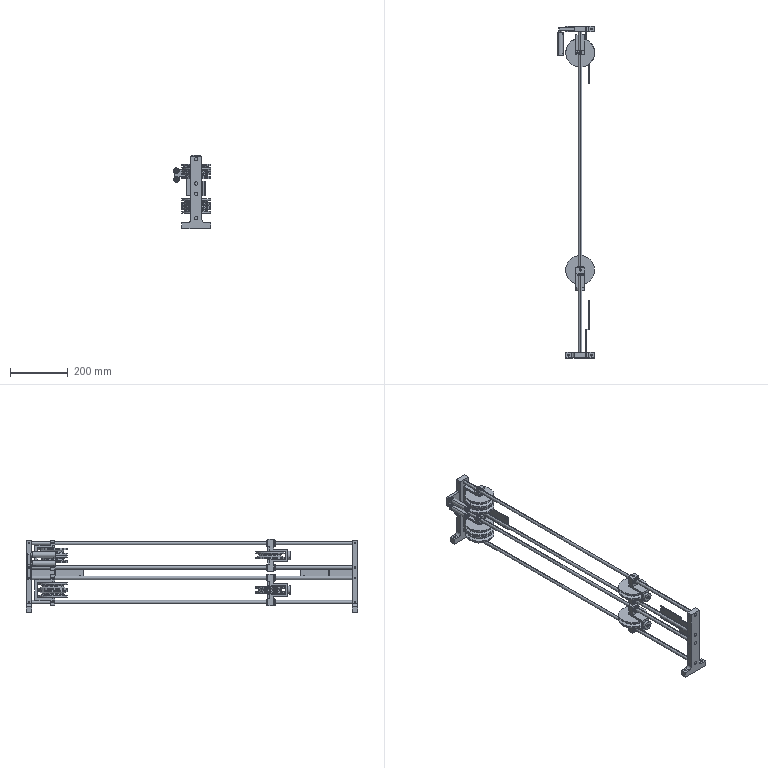Assembly | SolidWorks | mm | 77 component files | 77 solids | 2793 faces | box 129 x 1150 x 253 mm | volume 2246708 mm3 | cylinder 1288 | plane 521 | sphere 448 | torus 400 | cone 72 | spline 64 | commonest cylinder face diameters 1.794 x416 8 x72 12 x52 22 x48 12.2 x48 19.3 x48 2 x48 4.2 x40
Bill of materials:
B606ZZ | 4 |  | Short thick annular ring with a central through bore and a thin concentric recessed groove on the end face between the inner and outer diameters; edges slightly rounded.
GB_T894-2017[RetainingRingForShaftA-type(d0_9)6] | 2 |  | Flat, thin open ring split at one point, with two small lugs next to the gap, each having a round hole.
JL001-03-06-001 | 2 |  | Stepped cylindrical shaft: a long slender shank with a chamfered end, a short larger-diameter collar near the other end, then a reduced neck and a short end journal.
JL001-03-06-002 | 2 |  | Plain straight round tube with a concentric through bore and square-cut ends.
JL001-05-01-001 | 2 |  | Inverted-T bracket: a tall rectangular upright on a wider base flange, joined by fillets. The upright has four round through holes in its main face and four small holes in its narrow edge face; the base flange has one hole at each end.
JL001-05-01-002 | 4 |  | Very slender solid round rod of constant diameter with plain ends.
JL001-05-01-010 | 2 |  | Thin flat strip with a joggle (Z-shaped offset bend) in the middle, so the two end sections lie in parallel offset planes. Each end has two round holes, and the holes at one end are larger than at the other.
JL001-05-01-011 | 1 |  | Thick flat plate shaped like an inverted L/hook: a wide head with a filleted inner notch and a long leg. Two through holes in the head's face, two holes in the narrow edge of the leg, and chamfered corners on the head.
B608ZZ | 12 |  | Short thick annular ring with a central bore and thin concentric grooves on the end face, one near the outer edge and one near the bore. Visually very similar to the first ring part.
JL001-05-01-003 | 2 |  | C-shaped bracket: two parallel arms joined by a back web. Each arm ends in a block with a large bore, split by a slot that runs to the edge, plus smaller holes, pockets and cross-holes.
JL001-05-01-004 | 6 |  | Disc-shaped pulley/sheave with two flanges and a circumferential groove between them (straight tapered flanks, rounded root), and a central through bore with a step or chamfer.
JL001-05-01-005 | 2 |  | Solid cylindrical pin with small chamfers at both ends.
JL001-05-01-006 | 10 |  | Flat annular ring (washer-like): a short cylinder with a large concentric through bore and plain flat faces.
JL001-05-01-013 | 4 |  | Rectangular bar block with roughly square cross-section. Two cylindrical through holes cross one long face near each end, and a semicircular groove runs through the full height of the opposite long face at mid-length.
GB_T894-2017[RetainingRingForShaftA-type(d0_10)21] | 8 |  | Thin flat split ring with an open gap. Each end next to the gap has a widened lug with a small round hole, so it looks like a retaining-ring-style profile.
JL001-05-01-007 | 2 |  | Bracket-like block with a stepped C/Z-shaped side profile. Two end blocks are offset, and each has a large through bore. Several small holes are also visible: one central small hole, small holes on the end-block faces, and a small hole on the side of the central web.
JL001-05-01-008 | 2 |  | Slender solid cylindrical pin with small chamfers or edge breaks at both ends.
JL001-05-01-009 | 2 |  | Thick disc or spacer with a small concentric through hole. Its thickness is a sizable fraction of its diameter.
JL001-05-01-012 | 4 |  | Rectangular block with a semicircular groove running the full height of one long face at mid-length. Two cylindrical through holes, one on each side of the groove, pass through the same face.
LM12UU | 4 |  | Thick-walled hollow cylindrical sleeve with a plain through-bore and two shallow circumferential grooves on the outside, one near each end. Small spherical elements show inside the bore, arranged in axial rows. The overall shape looks like a linear ball bushing.
Mates:
1. coincident | JL001-05-01-001-1 face at (0, -10, 0) dir (0, -1, 0) | JL001-05-01-002-1 face at (0, -10, 105) dir (0, -1, 0)
2. coincident | JL001-05-01-001-1 face at (0, -10, 0) dir (0, -1, 0) | JL001-05-01-002-2 face at (0, -10, 21) dir (0, -1, 0)
3. coincident | JL001-05-01-001-1 face at (0, -10, 0) dir (0, -1, 0) | JL001-05-01-002-3 face at (0, -10, -15) dir (0, -1, 0)
4. coincident | JL001-05-01-001-1 face at (0, -10, 0) dir (0, -1, 0) | JL001-05-01-002-4 face at (0, -10, -99) dir (0, -1, 0)
5. concentric | JL001-05-01-001-1 face at (0, 10, -99) dir (0, 1, 0) r 6 | JL001-05-01-002-4 face at (0, 1140, -99) dir (0, -1, 0) r 6
6. concentric | JL001-05-01-001-1 face at (0, 10, -15) dir (0, 1, 0) r 6 | JL001-05-01-002-3 face at (0, 1140, -15) dir (0, -1, 0) r 6
7. concentric | JL001-05-01-001-1 face at (0, 10, 21) dir (0, 1, 0) r 6 | JL001-05-01-002-2 face at (0, 1140, 21) dir (0, -1, 0) r 6
8. concentric | JL001-05-01-001-1 face at (0, 10, 105) dir (0, 1, 0) r 6 | JL001-05-01-002-1 face at (0, 1140, 105) dir (0, -1, 0) r 6
9. concentric | JL001-05-01-002-1 face at (0, 1140, 105) dir (0, -1, 0) r 6 | JL001-05-01-001-2 face at (0, 1140, 105) dir (0, 1, 0) r 6
10. concentric | JL001-05-01-002-4 face at (0, 1140, -99) dir (0, -1, 0) r 6 | JL001-05-01-001-2 face at (0, 1140, -99) dir (0, 1, 0) r 6
11. coincident | JL001-05-01-002-1 face at (0, 1140, 105) dir (0, 1, 0) | JL001-05-01-001-2 face at (0, 1140, 0) dir (0, 1, 0)
12. concentric | JL001-05-01-002-4 face at (0, 1140, -99) dir (0, -1, 0) r 6 | JL001-05-02-2/JL001-05-01-003-1 face at (0, 1040, -99) dir (0, -1, 0) r 6
13. concentric | JL001-05-01-002-2 face at (0, 1140, 21) dir (0, -1, 0) r 6 | JL001-05-02-1/JL001-05-01-003-1 face at (0, 1040, 21) dir (0, -1, 0) r 6
14. concentric | JL001-05-01-002-3 face at (0, 1140, -15) dir (0, -1, 0) r 6 | JL001-05-02-2/JL001-05-01-003-1 face at (0, 1040, -15) dir (0, -1, 0) r 6
15. concentric | JL001-05-01-002-1 face at (0, 1140, 105) dir (0, -1, 0) r 6 | JL001-05-02-1/JL001-05-01-003-1 face at (0, 1040, 105) dir (0, -1, 0) r 6
16. distance | JL001-05-02-2/JL001-05-01-003-1 face at (-15, 1040, -4.5) dir (0, -1, 0) | JL001-05-01-001-2 face at (0, 1120, 0) dir (0, -1, 0)
17. concentric | JL001-05-01-002-4 face at (0, 1140, -99) dir (0, -1, 0) r 6 | JL001-05-03-2/LM12UU-2 face at (0, 279.648, -99) dir (0, -1, 0) r 6.3
18. concentric | JL001-05-01-002-2 face at (0, 1140, 21) dir (0, -1, 0) r 6 | JL001-05-03-1/LM12UU-2 face at (0, 279.648, 21) dir (0, -1, 0) r 6.3
19. concentric | JL001-05-01-002-1 face at (0, 1140, 105) dir (0, -1, 0) r 6 | JL001-05-03-1/LM12UU-1 face at (0, 279.648, 105) dir (0, -1, 0) r 6.3
20. concentric | JL001-05-01-002-3 face at (0, 1140, -15) dir (0, -1, 0) r 6 | JL001-05-03-2/LM12UU-1 face at (0, 279.648, -15) dir (0, -1, 0) r 6.3
21. coincident | JL001-05-03-1/JL001-05-01-007-1 face at (15, 302.348, 118) dir (0, 1, 0) | JL001-05-03-2/JL001-05-01-007-1 face at (15, 302.348, -2) dir (0, 1, 0)
22. coincident | JL001-05-01-001-1 face at (20, 10, -115) dir (1, 0, 0) | JL001-05-01-010-1 face at (20, -10, 28) dir (-1, 0, 0)
23. concentric | JL001-05-01-001-1 face at (20, 0, 21) dir (1, 0, 0) r 2.1 | JL001-05-01-010-1 face at (22, 0, 21) dir (1, 0, 0) r 2.75
24. concentric | JL001-05-01-001-1 face at (20, 0, -15) dir (1, 0, 0) r 2.1 | JL001-05-01-010-1 face at (22, 0, -15) dir (1, 0, 0) r 2.75
25. coincident | JL001-05-01-001-2 face at (20, 1140, -115) dir (1, 0, 0) | JL001-05-01-010-2 face at (20, 1140, -22) dir (-1, 0, 0)
26. concentric | JL001-05-01-001-2 face at (20, 1130, -15) dir (1, 0, 0) r 2.1 | JL001-05-01-010-2 face at (22, 1130, -15) dir (1, 0, 0) r 2.75
27. concentric | JL001-05-01-001-2 face at (20, 1130, 21) dir (1, 0, 0) r 2.1 | JL001-05-01-010-2 face at (22, 1130, 21) dir (1, 0, 0) r 2.75
28. coincident | JL001-05-01-001-2 face at (-20, 1140, -115) dir (-1, 0, 0) | JL001-05-01-011-1 face at (-20, 1135, -20) dir (1, 0, 0)
29. concentric | JL001-05-01-001-2 face at (20, 1130, -15) dir (1, 0, 0) r 2.1 | JL001-05-01-011-1 face at (-35, 1130, -15) dir (-1, 0, 0) r 2.75
30. concentric | JL001-05-01-011-1 face at (-69, 1135, 65) dir (0, 1, 0) r 3 | JL001-03-06-1/JL001-03-06-001-1 face at (-69, 1135, 65) dir (0, 1, 0) r 3
31. coincident | JL001-05-01-011-1 face at (-47.5, 1125, 25) dir (0, -1, 0) | JL001-03-06-1/JL001-03-06-001-1 face at (-64.814, 1125, 67.735) dir (0, 1, 0)
32. concentric | JL001-05-01-011-1 face at (-69, 1135, 35) dir (0, 1, 0) r 3 | JL001-03-06-2/JL001-03-06-001-1 face at (-69, 1135, 35) dir (0, 1, 0) r 3
33. coincident | JL001-05-01-011-1 face at (-47.5, 1125, 25) dir (0, -1, 0) | JL001-03-06-2/JL001-03-06-001-1 face at (-64.814, 1125, 37.735) dir (0, 1, 0)
34. concentric | JL001-05-01-001-2 face at (20, 1130, 21) dir (1, 0, 0) r 2.1 | JL001-05-01-011-1 face at (-35, 1130, 21) dir (-1, 0, 0) r 2.75
35. coincident | JL001-05-02-1/JL001-05-01-003-1 face at (-15, 1040, 115.5) dir (0, -1, 0) | JL001-05-02-2/JL001-05-01-003-1 face at (-15, 1040, -4.5) dir (0, -1, 0)
36. concentric | JL001-03-06-001-1 face at (0, 0, 0) dir (0, -1, 0) r 3 | B606ZZ-1 face at (0, 20.3, 0) dir (0, 1, 0) r 3
37. coincident | JL001-03-06-001-1 face at (3, 20, 0) dir (0, 1, 0) | B606ZZ-1 face at (3.3, 20, 0) dir (0, -1, 0)
38. concentric | B606ZZ-1 face at (0, 20.3, 0) dir (0, 1, 0) r 8.5 | JL001-03-06-002-1 face at (0, 98, 0) dir (0, 1, 0) r 8.5
39. coincident | B606ZZ-1 face at (8.2, 26, 0) dir (0, 1, 0) | JL001-03-06-002-1 face at (8.5, 26, 0) dir (0, -1, 0)
40. concentric | JL001-03-06-001-1 face at (0, 0, 0) dir (0, -1, 0) r 3 | B606ZZ-2 face at (0, 90.3, 0) dir (0, 1, 0) r 3
41. coincident | JL001-03-06-002-1 face at (7, 90, 0) dir (0, 1, 0) | B606ZZ-2 face at (7.5, 90, 0) dir (0, -1, 0)
42. concentric | JL001-03-06-001-1 face at (0, 0, 0) dir (0, -1, 0) r 2.85 | GB_T894-2017[RetainingRingForShaftA-type(d0_9)6]-1 face at (0, 96, 0) dir (0, 1, 0) r 2.85
43. coincident | JL001-03-06-001-1 face at (2.85, 96, 0) dir (0, 1, 0) | GB_T894-2017[RetainingRingForShaftA-type(d0_9)6]-1 face at (0.7354, 96, 4.114) dir (0, -1, 0)
44. concentric | JL001-05-01-003-1 face at (-52.5, 27.5, 0) dir (-1, 0, 0) r 4 | JL001-05-01-005-1 face at (-34, 27.5, 0) dir (1, 0, 0) r 4
45. width | JL001-05-01-005-1 face at (-34, 27.5, 0) dir (-1, 0, 0) | JL001-05-01-005-1 face at (34, 27.5, 0) dir (1, 0, 0) | JL001-05-01-003-1 face at (-27, 97, -15) dir (1, 0, 0) | JL001-05-01-003-1 face at (27, 97, -15) dir (-1, 0, 0)
46. concentric | JL001-05-01-004-2 face at (-13, 27.5, 0) dir (1, 0, 0) r 11 | B608ZZ-2 face at (-1.3, 27.5, 0) dir (-1, 0, 0) r 11
47. concentric | JL001-05-01-004-2 face at (-13, 27.5, 0) dir (1, 0, 0) r 11 | B608ZZ-1 face at (-18.3, 27.5, 0) dir (-1, 0, 0) r 11
48. coincident | JL001-05-01-004-2 face at (-18, 16.5, 0) dir (-1, 0, 0) | B608ZZ-1 face at (-18, 37.15, 0) dir (1, 0, 0)
49. coincident | JL001-05-01-004-2 face at (-8, 18.5, 0) dir (1, 0, 0) | B608ZZ-2 face at (-8, 38.2, 0) dir (-1, 0, 0)
50. concentric | JL001-05-01-004-1 face at (13, 27.5, 0) dir (1, 0, 0) r 11 | B608ZZ-3 face at (24.7, 27.5, 0) dir (-1, 0, 0) r 11
51. coincident | JL001-05-01-004-1 face at (18, 18.581, -1.208) dir (1, 0, 0) | B608ZZ-3 face at (18, 38.2, 0) dir (-1, 0, 0)
52. concentric | JL001-05-01-004-1 face at (13, 27.5, 0) dir (1, 0, 0) r 11 | B608ZZ-4 face at (7.7, 27.5, 0) dir (-1, 0, 0) r 11
53. coincident | JL001-05-01-004-1 face at (8, 16.6, -1.477) dir (-1, 0, 0) | B608ZZ-4 face at (8, 37.15, 0) dir (1, 0, 0)
54. concentric | JL001-05-01-005-1 face at (-34, 27.5, 0) dir (1, 0, 0) r 4 | JL001-05-01-006-1 face at (-25, 27.5, 0) dir (-1, 0, 0) r 4.05
55. coincident | JL001-05-01-003-1 face at (-27, 97, -15) dir (1, 0, 0) | JL001-05-01-006-1 face at (-27, 27.5, 0) dir (-1, 0, 0)
56. concentric | JL001-05-01-005-1 face at (-34, 27.5, 0) dir (1, 0, 0) r 4 | JL001-05-01-006-2 face at (1, 27.5, 0) dir (-1, 0, 0) r 4.05
57. concentric | JL001-05-01-005-1 face at (-34, 27.5, 0) dir (1, 0, 0) r 4 | JL001-05-01-006-3 face at (27, 27.5, 0) dir (-1, 0, 0) r 4.05
58. coincident | JL001-05-01-003-1 face at (27, 97, -15) dir (-1, 0, 0) | JL001-05-01-006-3 face at (27, 27.5, 0) dir (1, 0, 0)
59. concentric | JL001-05-01-005-1 face at (-34, 27.5, 0) dir (1, 0, 0) r 4 | B608ZZ-1 face at (-18.3, 27.5, 0) dir (-1, 0, 0) r 4
60. coincident | B608ZZ-2 face at (-1, 31.8, 0) dir (1, 0, 0) | JL001-05-01-006-2 face at (-1, 27.5, 0) dir (-1, 0, 0)
61. concentric | JL001-05-01-005-1 face at (-34, 27.5, 0) dir (1, 0, 0) r 4 | B608ZZ-3 face at (24.7, 27.5, 0) dir (-1, 0, 0) r 4
62. coincident | B608ZZ-4 face at (1, 33.6, 0) dir (-1, 0, 0) | JL001-05-01-006-2 face at (1, 27.5, 0) dir (1, 0, 0)
63. width | B608ZZ-3 face at (25, 31.8, 0) dir (1, 0, 0) | B608ZZ-1 face at (-25, 38.2, 0) dir (-1, 0, 0) | JL001-05-01-003-1 face at (-27, 97, -15) dir (1, 0, 0) | JL001-05-01-003-1 face at (27, 97, -15) dir (-1, 0, 0)
64. concentric | JL001-05-01-005-1 face at (-34, 27.5, 0) dir (1, 0, 0) r 4 | JL001-05-01-013-1 face at (-35, 27.5, 0) dir (-1, 0, 0) r 4
65. concentric | JL001-05-01-005-1 face at (-34, 27.5, 0) dir (1, 0, 0) r 4 | JL001-05-01-013-2 face at (27, 27.5, 0) dir (-1, 0, 0) r 4
66. concentric | JL001-05-01-003-1 face at (31, 27.5, -10) dir (0, 1, 0) r 1.65 | JL001-05-01-013-2 face at (31, 35, -10) dir (0, 1, 0) r 2.25
67. concentric | JL001-05-01-003-1 face at (-31, 27.5, -10) dir (0, 1, 0) r 1.65 | JL001-05-01-013-1 face at (-31, 35, -10) dir (0, 1, 0) r 2.25
68. concentric | JL001-05-01-007-1 face at (-55, 27.5, 0) dir (-1, 0, 0) r 4 | JL001-05-01-008-1 face at (-29, 27.5, 0) dir (1, 0, 0) r 4
69. width | JL001-05-01-008-1 face at (-29, 27.5, 0) dir (-1, 0, 0) | JL001-05-01-008-1 face at (29, 27.5, 0) dir (1, 0, 0) | JL001-05-01-007-1 face at (-14, 97, -15) dir (1, 0, 0) | JL001-05-01-007-1 face at (14, 97, -15) dir (-1, 0, 0)
70. concentric | JL001-05-01-004-1 face at (0, 27.5, 0) dir (1, 0, 0) r 11 | B608ZZ-3 face at (11.7, 27.5, 0) dir (-1, 0, 0) r 11
71. coincident | JL001-05-01-004-1 face at (5, 18.518, 0.5632) dir (1, 0, 0) | B608ZZ-3 face at (5, 38.2, 0) dir (-1, 0, 0)
72. concentric | JL001-05-01-004-1 face at (0, 27.5, 0) dir (1, 0, 0) r 11 | B608ZZ-4 face at (-5.3, 27.5, 0) dir (-1, 0, 0) r 11
73. coincident | JL001-05-01-004-1 face at (-5, 16.522, 0.6884) dir (-1, 0, 0) | B608ZZ-4 face at (-5, 37.15, 0) dir (1, 0, 0)
74. concentric | JL001-05-01-008-1 face at (-29, 27.5, 0) dir (1, 0, 0) r 4 | JL001-05-01-006-1 face at (-12, 27.5, 0) dir (-1, 0, 0) r 4.05
75. coincident | JL001-05-01-007-1 face at (-14, 97, -15) dir (1, 0, 0) | JL001-05-01-006-1 face at (-14, 27.5, 0) dir (-1, 0, 0)
76. concentric | JL001-05-01-008-1 face at (-29, 27.5, 0) dir (1, 0, 0) r 4 | JL001-05-01-006-3 face at (14, 27.5, 0) dir (-1, 0, 0) r 4.05
77. coincident | JL001-05-01-007-1 face at (14, 97, -15) dir (-1, 0, 0) | JL001-05-01-006-3 face at (14, 27.5, 0) dir (1, 0, 0)
78. concentric | JL001-05-01-008-1 face at (-29, 27.5, 0) dir (1, 0, 0) r 4 | B608ZZ-3 face at (11.7, 27.5, 0) dir (-1, 0, 0) r 4
79. width | JL001-05-01-004-1 face at (12, 16.522, 0.6884) dir (1, 0, 0) | JL001-05-01-004-1 face at (-12, -22.402, 3.129) dir (-1, 0, 0) | JL001-05-01-007-1 face at (14, 97, -15) dir (-1, 0, 0) | JL001-05-01-007-1 face at (-14, 97, -15) dir (1, 0, 0)
80. concentric | JL001-05-01-007-1 face at (-42, 35, 0) dir (0, 1, 0) r 10.5 | LM12UU-1 face at (-42, 12.3, 0) dir (0, -1, 0) r 10.5
81. concentric | JL001-05-01-007-1 face at (42, 35, 0) dir (0, 1, 0) r 10.5 | LM12UU-2 face at (42, 12.3, 0) dir (0, -1, 0) r 10.5
82. coincident | JL001-05-01-007-1 face at (-55, 35, 15) dir (0, 1, 0) | LM12UU-2 face at (42, 35, 10.5) dir (0, 1, 0)
83. coincident | JL001-05-01-007-1 face at (-55, 35, 15) dir (0, 1, 0) | LM12UU-1 face at (-42, 35, 10.5) dir (0, 1, 0)
84. coincident | LM12UU-1 face at (-42, 14.6, 10.5) dir (0, -1, 0) | GB_T894-2017[RetainingRingForShaftA-type(d0_10)21]-3 face at (-50.803, 14.6, 8.554) dir (0, 1, 0)
85. coincident | LM12UU-1 face at (-42, 35, 10.5) dir (0, 1, 0) | GB_T894-2017[RetainingRingForShaftA-type(d0_10)21]-2 face at (-50.803, 35, -8.554) dir (0, -1, 0)
86. coincident | LM12UU-2 face at (42, 35, 10.5) dir (0, 1, 0) | GB_T894-2017[RetainingRingForShaftA-type(d0_10)21]-1 face at (33.197, 35, -8.554) dir (0, -1, 0)
87. coincident | LM12UU-2 face at (42, 14.6, 10.5) dir (0, -1, 0) | GB_T894-2017[RetainingRingForShaftA-type(d0_10)21]-4 face at (33.197, 14.6, 8.554) dir (0, 1, 0)
88. concentric | LM12UU-2 face at (42, 12.3, 0) dir (0, -1, 0) r 10 | GB_T894-2017[RetainingRingForShaftA-type(d0_10)21]-4 face at (42, 14.6, 0) dir (0, -1, 0) r 10.05
89. concentric | LM12UU-2 face at (42, 12.3, 0) dir (0, -1, 0) r 10 | GB_T894-2017[RetainingRingForShaftA-type(d0_10)21]-1 face at (42, 35, 0) dir (0, 1, 0) r 10.05
90. concentric | LM12UU-1 face at (-42, 12.3, 0) dir (0, -1, 0) r 10 | GB_T894-2017[RetainingRingForShaftA-type(d0_10)21]-2 face at (-42, 35, 0) dir (0, 1, 0) r 10.05
91. concentric | LM12UU-1 face at (-42, 12.3, 0) dir (0, -1, 0) r 10 | GB_T894-2017[RetainingRingForShaftA-type(d0_10)21]-3 face at (-42, 14.6, 0) dir (0, -1, 0) r 10.05
92. coincident | JL001-05-01-007-1 face at (-55, -35, 15) dir (0, -1, 0) | JL001-05-01-009-1 face at (0, -35, 0) dir (0, 1, 0)
93. concentric | JL001-05-01-007-1 face at (0, -35, 0) dir (0, -1, 0) r 2.5 | JL001-05-01-009-1 face at (0, -45, 0) dir (0, 1, 0) r 15
94. concentric | JL001-05-01-008-1 face at (-29, 27.5, 0) dir (1, 0, 0) r 4 | JL001-05-01-012-2 face at (14, 27.5, 0) dir (1, 0, 0) r 4
95. concentric | JL001-05-01-008-1 face at (-29, 27.5, 0) dir (1, 0, 0) r 4 | JL001-05-01-012-1 face at (-30, 27.5, 0) dir (1, 0, 0) r 4
96. concentric | JL001-05-01-007-1 face at (22, 27.5, -9) dir (0, 1, 0) r 1.65 | JL001-05-01-012-2 face at (22, 35, -9) dir (0, 1, 0) r 2.25
97. concentric | JL001-05-01-007-1 face at (-22, 27.5, 9) dir (0, 1, 0) r 1.65 | JL001-05-01-012-1 face at (-22, 35, 9) dir (0, 1, 0) r 2.25